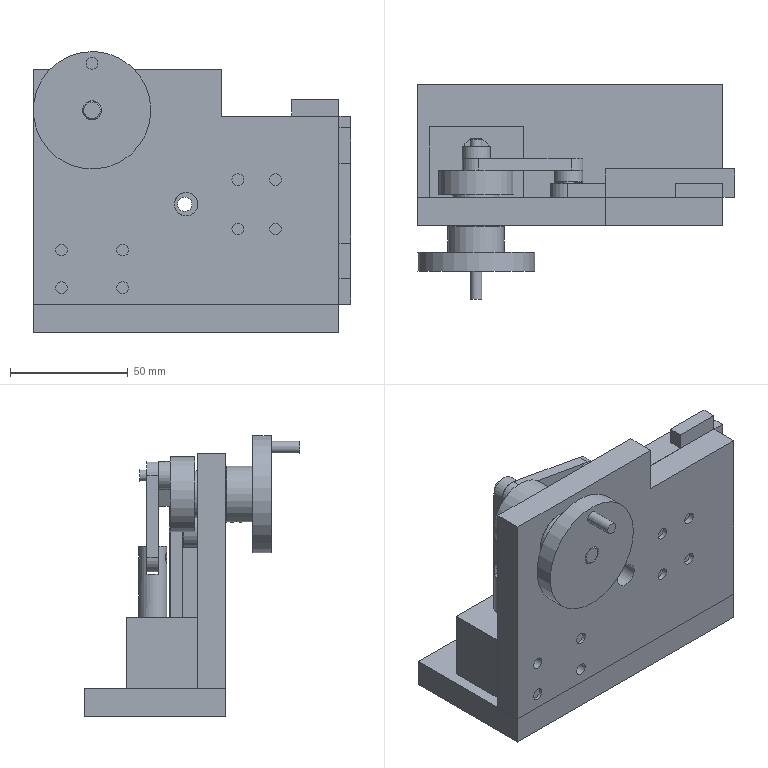Assembly | NX | mm | 26 component files | 26 solids | 254 faces | box 135 x 91.5 x 119.5 mm | volume 357094 mm3 | plane 168 | cylinder 80 | cone 6 | commonest cylinder face diameters 5 x35 12 x9 5.5 x8 10 x7 5.1 x6 8.28 x4 8 x2 6.1 x2
Bill of materials:
unnamed part 1 | 1 |  | Thick plate-like block with a stepped profile: a raised rectangular pad on one face with four round holes in a 2x2 pattern, with rectangular steps/recesses along the edges.
unnamed part 2 | 1 |  | Flat plate of constant thickness with two V-shaped notches cut into one long edge, giving a sawtooth edge.
unnamed part 3 | 6 |  | Plain solid cylinder (rod) with flat ends, roughly 2.5-3 times as long as its diameter.
unnamed part 4 | 2 |  | Stepped cylindrical pin: a short, larger-diameter head and a longer, smaller-diameter shank on the same axis.
unnamed part 5 | 1 |  | Rectangular block with one larger round hole in the top face and four smaller round holes in a rectangular pattern on one side face.
unnamed part 6 | 1 |  | Flanged hub: a circular flange disc with a smaller cylindrical boss on one side, a central through hole, and one small offset hole near the flange rim.
unnamed part 7 | 1 |  | Flat bar or link with one rounded end carrying a round through hole and a pointed (chevron) tip at the other end.
unnamed part 8 | 3 |  | Short plain solid cylinder with flat ends, slightly longer than its diameter.
unnamed part 9 | 1 |  | Cylindrical body with a conical pointed top and a rectangular notch cut into the bottom edge of the cylindrical wall. There is a small diameter step on the lower section.
unnamed part 10 | 1 |  | Flat plate with a rectangular step cut from one corner, two larger round holes, and eight smaller round holes arranged in two 2x2 groups.
unnamed part 11 | 1 |  | Cylindrical rod with a slotted (forked) end: a rectangular slot across one end and a cross hole through the forked portion, perpendicular to the slot. The slotted end looks slightly smaller in diameter.
unnamed part 12 | 1 |  | Rectangular flat plate with one larger round hole and two smaller round holes, all near one long edge.
unnamed part 13 | 1 |  | Long, thin, flat bar with one fully rounded end and one square end. It has a row of through-features along its centerline: a small round hole near the rounded end, an elongated obround slot, a larger round hole, and a slot that is open at the square end and has a rounded inner end.
unnamed part 14 | 1 |  | Stepped turned part shaped like a shaft. It has a large-diameter disc flange, a thin, slightly smaller step or boss on one face of the flange, a middle-diameter shaft section, and a smaller-diameter end shaft with a chamfered tip. A small round hole is set off-center in the flange, away from the axis.
unnamed part 15 | 1 |  | Flat link plate with rounded ends and two round through-holes, one near each end. The holes are different sizes, and the end around the larger hole looks wider, so the plate tapers slightly along its length.
unnamed part 16 | 2 |  | Plain cylindrical pin with a short cylindrical head of larger diameter at one end. The opposite end is flat.
unnamed part 17 | 1 |  | Flat, obround link plate with fully rounded ends and two equal-size round through-holes, one centered near each end.
Mates:
1. touch align | groove_guide_block 1 face | vertical_plate 1 face
2. touch align | groove_guide_block 1 edge | vertical_plate 1 edge
3. concentric | groove_guide_block 1 edge | vertical_plate 1 edge
4. fix | vertical_plate 1 component
5. concentric | short_link 1 edge | slide_rod 1 edge
6. fix | round_guide_block 1 component
7. parallel | long_link 1 face | bi_link 1 face
8. concentric | long_link 1 edge | bi_link 1 edge
9. fix | eccentric_wheel 1 component
10. concentric | long_link 1 edge | eccentric_wheel 1 edge
11. touch align | handwheel 1 face | eccentric_wheel 1 face
12. concentric | eccentric_wheel 1 edge | handwheel 1 edge
13. touch align | M5x6 1 face | eccentric_wheel 1 face
14. distance | M5x6 1 face | eccentric_wheel 1 face
15. touch align | round_guide_block 1 face | hex_screw_M5_35 1 face
16. concentric | round_guide_block 1 edge | hex_screw_M5_35 1 edge
17. touch align | hex_screw_M5_35 2 face | round_guide_block 1 face
18. concentric | round_guide_block 1 edge | hex_screw_M5_35 2 edge
19. touch align | hex_screw_M5_16 2 face | groove_guide_block 1 face
20. touch align | hex_screw_M5_16 1 face | groove_guide_block 1 face
21. concentric | hex_screw_M5_16 2 edge | groove_guide_block 1 edge
22. concentric | hex_screw_M5_16 1 edge | groove_guide_block 1 edge
23. distance | vertical_plate 1 edge | dowel_pin_5_20 4 face
24. distance | dowel_pin_5_20 5 face | vertical_plate 1 face
25. touch align | vertical_plate 1 face | dowel_pin_5_20 3 face
26. touch align | vertical_plate 1 face | dowel_pin_5_20 2 face
27. concentric | dowel_pin_5_20 3 edge | round_guide_block 1 edge
28. concentric | dowel_pin_5_20 2 edge | round_guide_block 1 edge
29. touch align | dowel_pin_5_12 3 face | slide_rod 1 face
30. distance | short_link 1 face | dowel_pin_5_12 3 face
31. fix | bi_link 1 component
32. touch align | tri_slider 1 face | groove_guide_block 1 face
33. touch align | vertical_plate 1 face | V_slider 1 face
34. touch align | V_slider 1 face | groove_guide_block 1 face
35. distance | V_slider 1 face | groove_guide_block 1 face
36. concentric | dowel_pin_5_20 1 edge | handwheel 1 edge